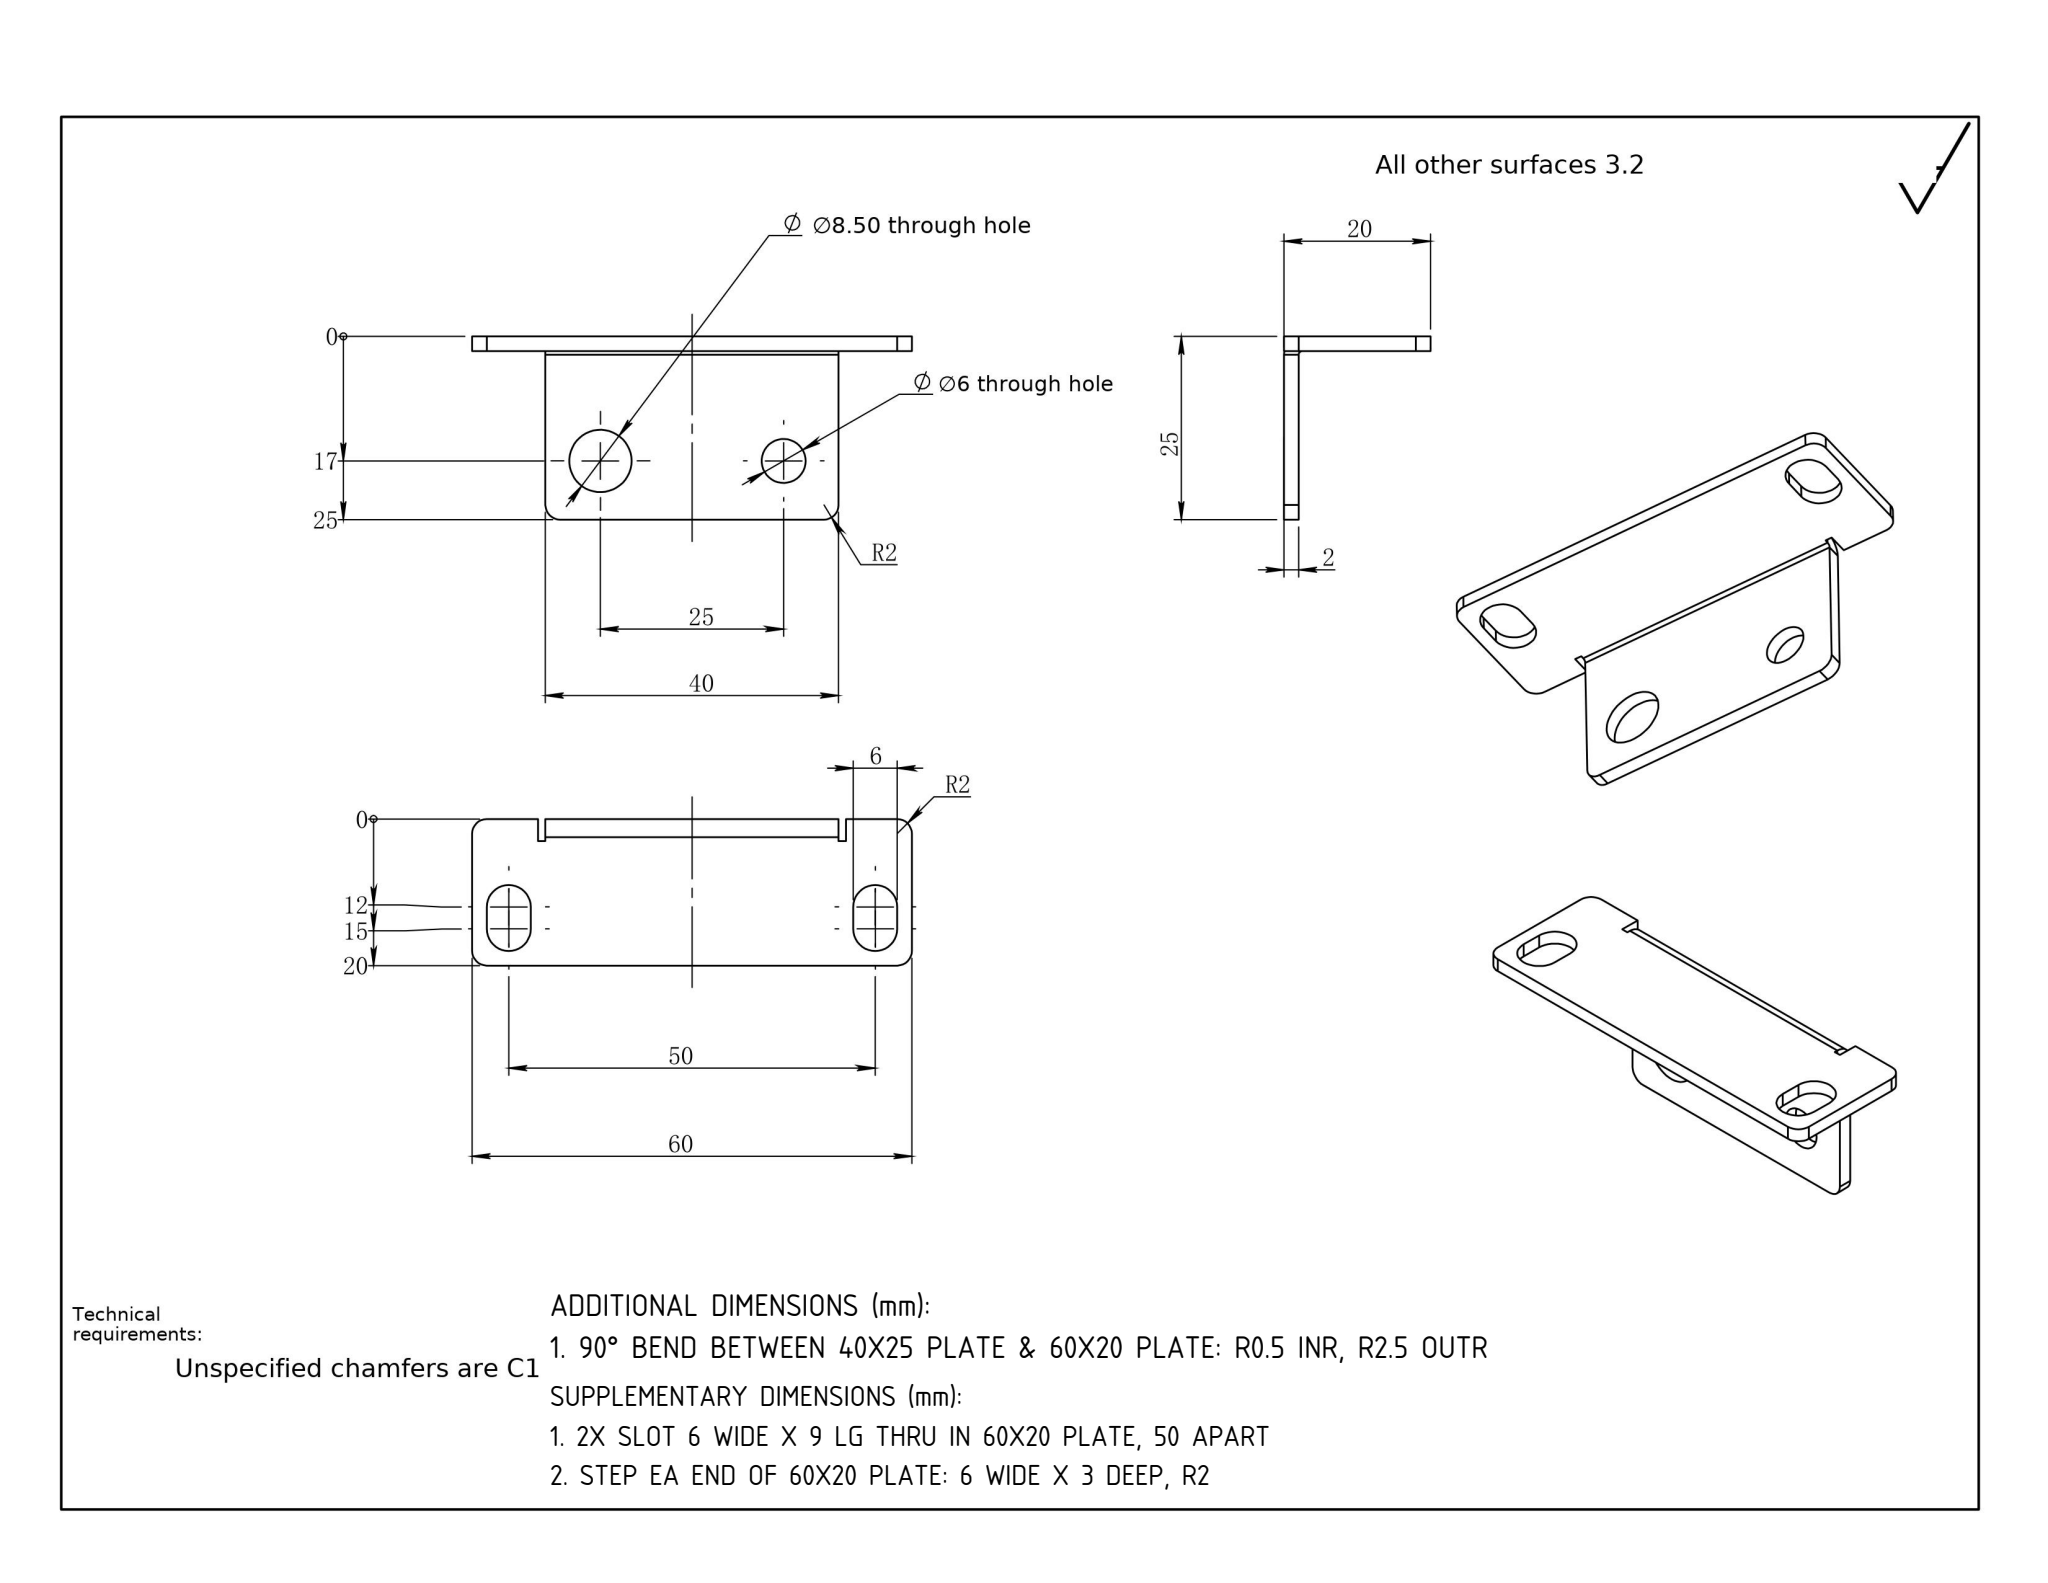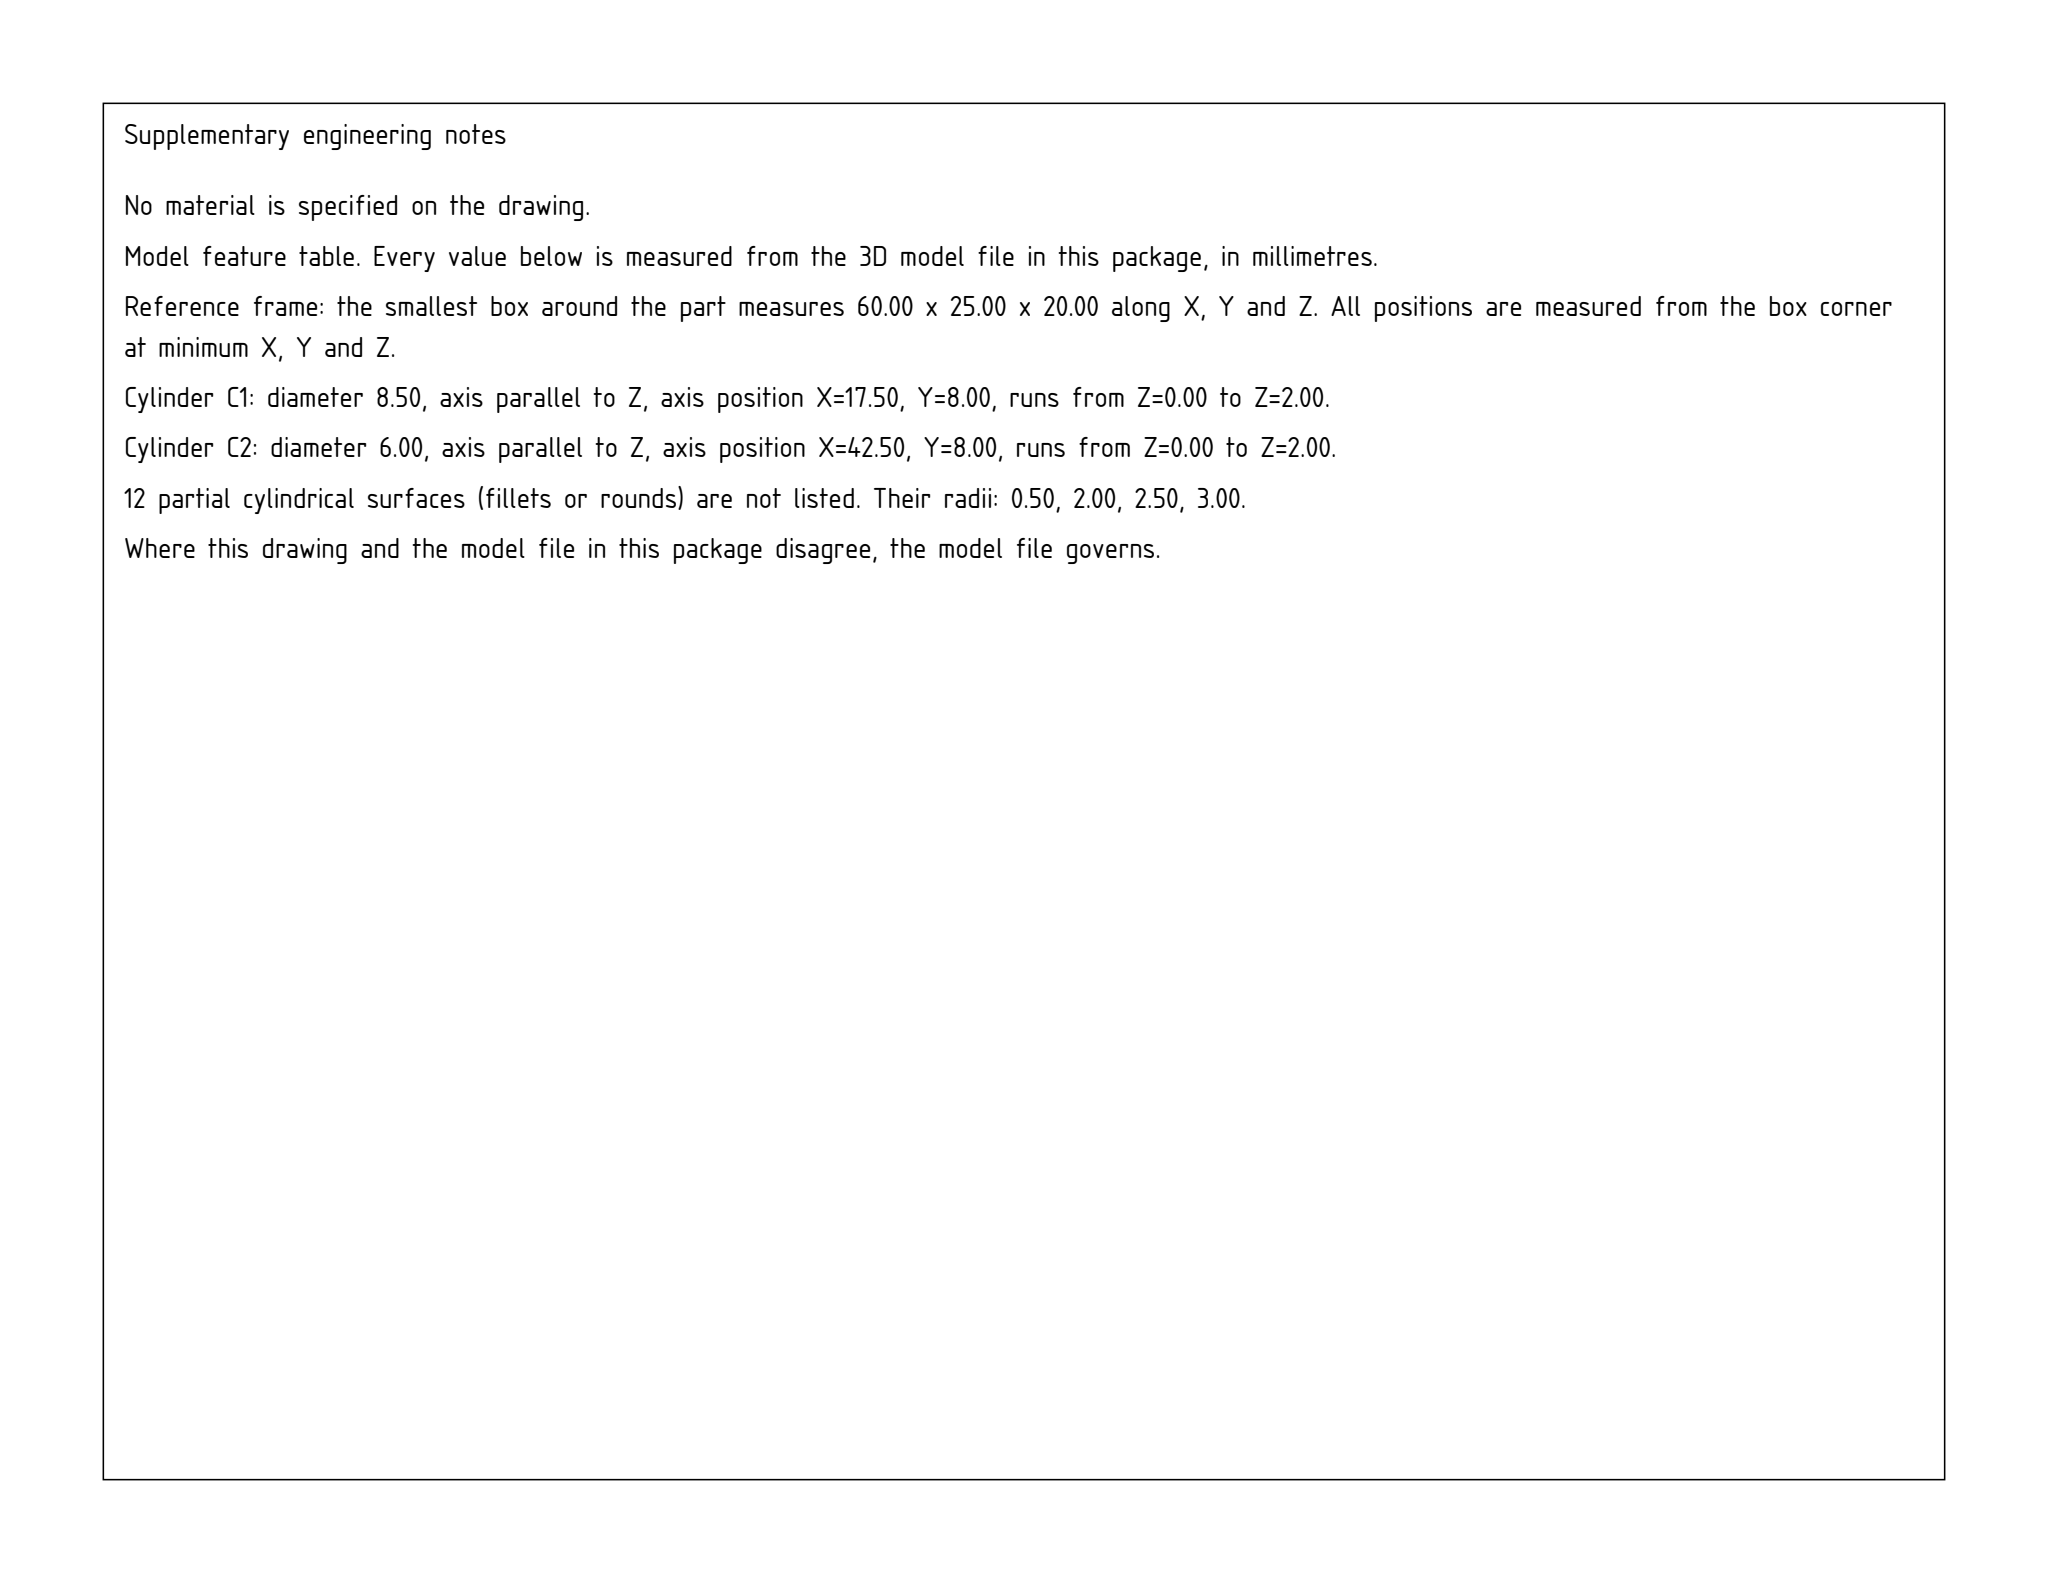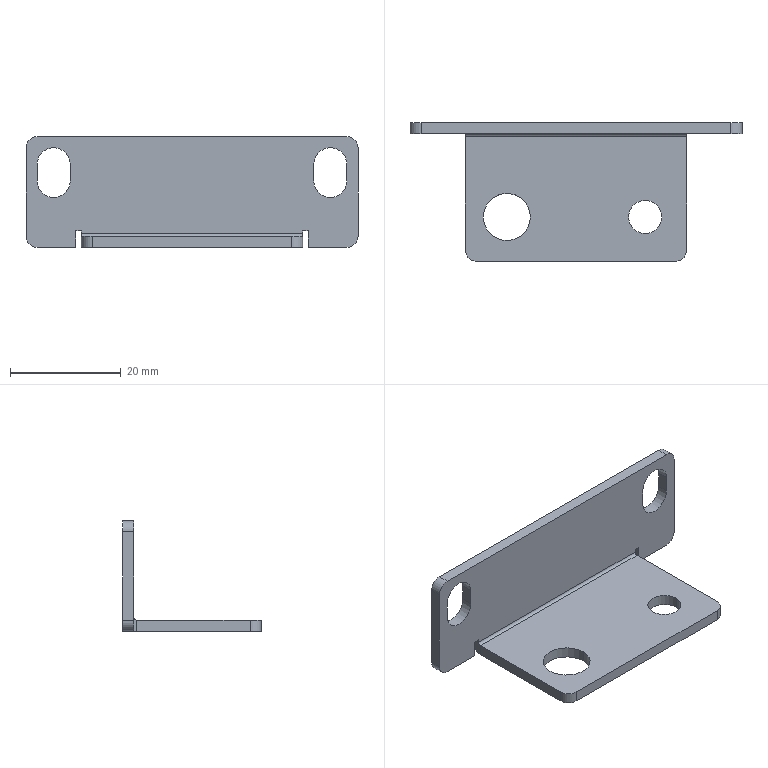Part | SolidWorks | mm | 1 solid | 40 faces | box 60 x 25 x 20 mm | volume 3811 mm3 | plane 24 | cylinder 16 | commonest cylinder face diameters 6 x6 4 x6 8.5 x2 5 x1 1 x1